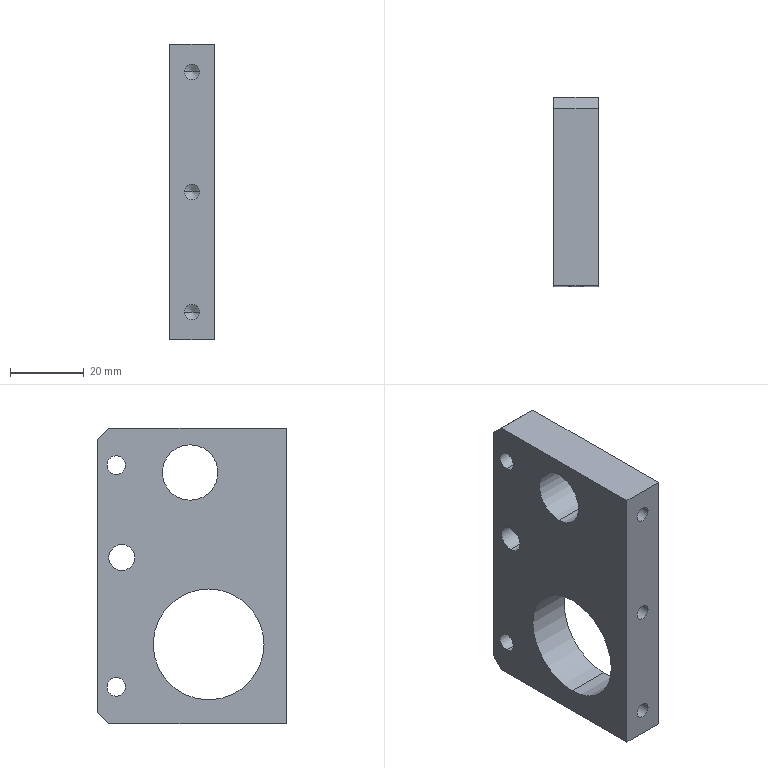Component | SolidWorks | A039-1 | 1 solid | 30 faces | box 12 x 51 x 80 mm | volume 36883 mm3 | cylinder 16 | plane 8 | cone 6 | commonest cylinder face diameters 4.2 x6 5 x4 7 x2 30 x2 15 x2
build123d program:
from build123d import *

# Parameters (mm, degrees)
SKETCH1_W             = 80
SKETCH1_H             = 51
BOSS_EXTRUDE1_DEPTH   = 12
CHAMFER1_SIZE         = 3
M5_TAPPED_HOLE1_D     = 4.2
M5_TAPPED_HOLE1_DEPTH = 10
M5_TAPPED_HOLE1_TIP   = 1.262
SKETCH6_R             = 7.5
SKETCH6_R_2           = 15
CUT_EXTRUDE1_DEPTH    = 20
M5_TAPPED_HOLE2_D     = 4.2
M5_TAPPED_HOLE2_DEPTH = 10
M5_TAPPED_HOLE2_TIP   = 1.262
M5_TAPPED_HOLE3_D     = 5
M8X1_0_TAPPED_HOLE1_D = 7


with BuildPart() as part:
    # Sketch1 → Boss-Extrude1 (new body)
    with BuildSketch(Plane.XY):
        Rectangle(SKETCH1_W, SKETCH1_H)
    extrude(amount=BOSS_EXTRUDE1_DEPTH)

    # Chamfer1
    chamfer1_edges = [part.edges().sort_by_distance(p)[0] for p in [
        (-40, 25.5, 6),
        (40, 25.5, 6),
    ]]
    chamfer(chamfer1_edges, length=CHAMFER1_SIZE)

    # M5 Tapped Hole1
    with Locations(Plane(origin=(0, -25.5, 0), x_dir=(-1, 0, 0), z_dir=(0, -1, 0))):
        with Locations((32.5, -6), (-32.5, -6)):
            Hole(M5_TAPPED_HOLE1_D / 2, depth=M5_TAPPED_HOLE1_DEPTH)
            with Locations((0, 0, -(M5_TAPPED_HOLE1_DEPTH + M5_TAPPED_HOLE1_TIP / 2))):  # 118° drill point
                Cone(0, M5_TAPPED_HOLE1_D / 2, M5_TAPPED_HOLE1_TIP, mode=Mode.SUBTRACT)

    # Sketch6 → Cut-Extrude1 (cut)
    with BuildSketch(Plane(origin=(0, 0, 0), x_dir=(-1, 0, 0), z_dir=(0, 0, -1))):
        with Locations((28, 0.5)):
            Circle(SKETCH6_R)
        with Locations((-18.5, -4.5)):
            Circle(SKETCH6_R_2)
    extrude(amount=-CUT_EXTRUDE1_DEPTH, mode=Mode.SUBTRACT)

    # M5 Tapped Hole2
    with Locations(Plane(origin=(0, -25.5, 0), x_dir=(-1, 0, 0), z_dir=(0, -1, 0))):
        with Locations((0, -6)):
            Hole(M5_TAPPED_HOLE2_D / 2, depth=M5_TAPPED_HOLE2_DEPTH)
            with Locations((0, 0, -(M5_TAPPED_HOLE2_DEPTH + M5_TAPPED_HOLE2_TIP / 2))):  # 118° drill point
                Cone(0, M5_TAPPED_HOLE2_D / 2, M5_TAPPED_HOLE2_TIP, mode=Mode.SUBTRACT)

    # M5 Tapped Hole3 (through all)
    with Locations(Plane.XY.offset(12)):
        with Locations((30, 20.5), (-30, 20.5)):
            Hole(M5_TAPPED_HOLE3_D / 2)

    # M8x1.0 Tapped Hole1 (through all)
    with Locations(Plane.XY.offset(12)):
        with Locations((-5, 19)):
            Hole(M8X1_0_TAPPED_HOLE1_D / 2)


solid = part.part

# Placed as in the assembly
solid = solid.moved(Location((321.381, 25.5, 60), (0, 90, 0)))
STEP:
#1=COLOUR_RGB('',0.7922,0.8196,0.9333);
#2=FILL_AREA_STYLE_COLOUR('',#1);
#3=FILL_AREA_STYLE('',(#2));
#4=SURFACE_STYLE_FILL_AREA(#3);
#5=SURFACE_SIDE_STYLE('',(#4));
#6=SURFACE_STYLE_USAGE(.BOTH.,#5);
#7=PRESENTATION_STYLE_ASSIGNMENT((#6));
#8=CARTESIAN_POINT('',(12.653,1.752,2.697));
#9=VERTEX_POINT('',#8);
#10=CARTESIAN_POINT('',(12.653,1.752,2.421));
#11=VERTEX_POINT('',#10);
#12=CARTESIAN_POINT('',(12.653,1.752,2.559));
#13=DIRECTION('',(1.,-0.,0.));
#14=DIRECTION('',(0.,0.,-1.));
#15=AXIS2_PLACEMENT_3D('',#12,#13,#14);
#16=CIRCLE('',#15,0.1378);
#17=EDGE_CURVE('',#9,#11,#16,.T.);
#18=ORIENTED_EDGE('',*,*,#17,.F.);
#19=CARTESIAN_POINT('',(13.125,1.752,2.697));
#20=VERTEX_POINT('',#19);
#21=CARTESIAN_POINT('',(13.125,1.752,2.697));
#22=DIRECTION('',(1.,-0.,0.));
#23=VECTOR('',#22,39.37);
#24=LINE('',#21,#23);
#25=EDGE_CURVE('',#9,#20,#24,.T.);
#26=ORIENTED_EDGE('',*,*,#25,.T.);
#27=CARTESIAN_POINT('',(13.125,1.752,2.421));
#28=VERTEX_POINT('',#27);
#29=CARTESIAN_POINT('',(13.125,1.752,2.559));
#30=DIRECTION('',(1.,-0.,0.));
#31=DIRECTION('',(0.,0.,-1.));
#32=AXIS2_PLACEMENT_3D('',#29,#30,#31);
#33=CIRCLE('',#32,0.1378);
#34=EDGE_CURVE('',#20,#28,#33,.T.);
#35=ORIENTED_EDGE('',*,*,#34,.T.);
#36=CARTESIAN_POINT('',(13.125,1.752,2.421));
#37=DIRECTION('',(1.,-0.,0.));
#38=VECTOR('',#37,39.37);
#39=LINE('',#36,#38);
#40=EDGE_CURVE('',#11,#28,#39,.T.);
#41=ORIENTED_EDGE('',*,*,#40,.F.);
#42=EDGE_LOOP('',(#18,#26,#35,#41));
#43=FACE_OUTER_BOUND('',#42,.T.);
#44=CARTESIAN_POINT('',(13.125,1.752,2.559));
#45=DIRECTION('',(1.,-0.,0.));
#46=DIRECTION('',(0.,0.,-1.));
#47=AXIS2_PLACEMENT_3D('',#44,#45,#46);
#48=CYLINDRICAL_SURFACE('',#47,0.1378);
#49=ADVANCED_FACE('',(#43),#48,.F.);
#50=CARTESIAN_POINT('',(12.653,1.811,1.28));
#51=VERTEX_POINT('',#50);
#52=CARTESIAN_POINT('',(12.653,1.811,1.083));
#53=VERTEX_POINT('',#52);
#54=CARTESIAN_POINT('',(12.653,1.811,1.181));
#55=DIRECTION('',(1.,-0.,0.));
#56=DIRECTION('',(0.,0.,-1.));
#57=AXIS2_PLACEMENT_3D('',#54,#55,#56);
#58=CIRCLE('',#57,0.09843);
#59=EDGE_CURVE('',#51,#53,#58,.T.);
#60=ORIENTED_EDGE('',*,*,#59,.F.);
#61=CARTESIAN_POINT('',(13.125,1.811,1.28));
#62=VERTEX_POINT('',#61);
#63=CARTESIAN_POINT('',(13.125,1.811,1.28));
#64=DIRECTION('',(1.,-0.,0.));
#65=VECTOR('',#64,39.37);
#66=LINE('',#63,#65);
#67=EDGE_CURVE('',#51,#62,#66,.T.);
#68=ORIENTED_EDGE('',*,*,#67,.T.);
#69=CARTESIAN_POINT('',(13.125,1.811,1.083));
#70=VERTEX_POINT('',#69);
#71=CARTESIAN_POINT('',(13.125,1.811,1.181));
#72=DIRECTION('',(1.,-0.,0.));
#73=DIRECTION('',(0.,0.,-1.));
#74=AXIS2_PLACEMENT_3D('',#71,#72,#73);
#75=CIRCLE('',#74,0.09843);
#76=EDGE_CURVE('',#62,#70,#75,.T.);
#77=ORIENTED_EDGE('',*,*,#76,.T.);
#78=CARTESIAN_POINT('',(13.125,1.811,1.083));
#79=DIRECTION('',(1.,-0.,0.));
#80=VECTOR('',#79,39.37);
#81=LINE('',#78,#80);
#82=EDGE_CURVE('',#53,#70,#81,.T.);
#83=ORIENTED_EDGE('',*,*,#82,.F.);
#84=EDGE_LOOP('',(#60,#68,#77,#83));
#85=FACE_OUTER_BOUND('',#84,.T.);
#86=CARTESIAN_POINT('',(13.125,1.811,1.181));
#87=DIRECTION('',(1.,-0.,0.));
#88=DIRECTION('',(0.,0.,-1.));
#89=AXIS2_PLACEMENT_3D('',#86,#87,#88);
#90=CYLINDRICAL_SURFACE('',#89,0.09843);
#91=ADVANCED_FACE('',(#85),#90,.F.);
#92=CARTESIAN_POINT('',(12.653,1.811,3.642));
#93=VERTEX_POINT('',#92);
#94=CARTESIAN_POINT('',(12.653,1.811,3.445));
#95=VERTEX_POINT('',#94);
#96=CARTESIAN_POINT('',(12.653,1.811,3.543));
#97=DIRECTION('',(1.,-0.,0.));
#98=DIRECTION('',(0.,0.,-1.));
#99=AXIS2_PLACEMENT_3D('',#96,#97,#98);
#100=CIRCLE('',#99,0.09843);
#101=EDGE_CURVE('',#93,#95,#100,.T.);
#102=ORIENTED_EDGE('',*,*,#101,.F.);
#103=CARTESIAN_POINT('',(13.125,1.811,3.642));
#104=VERTEX_POINT('',#103);
#105=CARTESIAN_POINT('',(13.125,1.811,3.642));
#106=DIRECTION('',(1.,-0.,0.));
#107=VECTOR('',#106,39.37);
#108=LINE('',#105,#107);
#109=EDGE_CURVE('',#93,#104,#108,.T.);
#110=ORIENTED_EDGE('',*,*,#109,.T.);
#111=CARTESIAN_POINT('',(13.125,1.811,3.445));
#112=VERTEX_POINT('',#111);
#113=CARTESIAN_POINT('',(13.125,1.811,3.543));
#114=DIRECTION('',(1.,-0.,0.));
#115=DIRECTION('',(0.,0.,-1.));
#116=AXIS2_PLACEMENT_3D('',#113,#114,#115);
#117=CIRCLE('',#116,0.09843);
#118=EDGE_CURVE('',#104,#112,#117,.T.);
#119=ORIENTED_EDGE('',*,*,#118,.T.);
#120=CARTESIAN_POINT('',(13.125,1.811,3.445));
#121=DIRECTION('',(1.,-0.,0.));
#122=VECTOR('',#121,39.37);
#123=LINE('',#120,#122);
#124=EDGE_CURVE('',#95,#112,#123,.T.);
#125=ORIENTED_EDGE('',*,*,#124,.F.);
#126=EDGE_LOOP('',(#102,#110,#119,#125));
#127=FACE_OUTER_BOUND('',#126,.T.);
#128=CARTESIAN_POINT('',(13.125,1.811,3.543));
#129=DIRECTION('',(1.,-0.,0.));
#130=DIRECTION('',(0.,0.,-1.));
#131=AXIS2_PLACEMENT_3D('',#128,#129,#130);
#132=CYLINDRICAL_SURFACE('',#131,0.09843);
#133=ADVANCED_FACE('',(#127),#132,.F.);
#134=CARTESIAN_POINT('',(12.972,0.3937,2.362));
#135=VERTEX_POINT('',#134);
#136=CARTESIAN_POINT('',(12.806,0.3937,2.362));
#137=VERTEX_POINT('',#136);
#138=CARTESIAN_POINT('',(12.889,0.3937,2.362));
#139=DIRECTION('',(-0.,-1.,-0.));
#140=DIRECTION('',(-1.,0.,0.));
#141=AXIS2_PLACEMENT_3D('',#138,#139,#140);
#142=CIRCLE('',#141,0.08268);
#143=EDGE_CURVE('',#135,#137,#142,.T.);
#144=ORIENTED_EDGE('',*,*,#143,.F.);
#145=CARTESIAN_POINT('',(12.972,-0.,2.362));
#146=VERTEX_POINT('',#145);
#147=CARTESIAN_POINT('',(12.972,-0.,2.362));
#148=DIRECTION('',(-0.,-1.,-0.));
#149=VECTOR('',#148,39.37);
#150=LINE('',#147,#149);
#151=EDGE_CURVE('',#135,#146,#150,.T.);
#152=ORIENTED_EDGE('',*,*,#151,.T.);
#153=CARTESIAN_POINT('',(12.806,-0.,2.362));
#154=VERTEX_POINT('',#153);
#155=CARTESIAN_POINT('',(12.889,-0.,2.362));
#156=DIRECTION('',(-0.,-1.,-0.));
#157=DIRECTION('',(-1.,0.,0.));
#158=AXIS2_PLACEMENT_3D('',#155,#156,#157);
#159=CIRCLE('',#158,0.08268);
#160=EDGE_CURVE('',#146,#154,#159,.T.);
#161=ORIENTED_EDGE('',*,*,#160,.T.);
#162=CARTESIAN_POINT('',(12.806,-0.,2.362));
#163=DIRECTION('',(-0.,-1.,-0.));
#164=VECTOR('',#163,39.37);
#165=LINE('',#162,#164);
#166=EDGE_CURVE('',#137,#154,#165,.T.);
#167=ORIENTED_EDGE('',*,*,#166,.F.);
#168=EDGE_LOOP('',(#144,#152,#161,#167));
#169=FACE_OUTER_BOUND('',#168,.T.);
#170=CARTESIAN_POINT('',(12.889,-0.,2.362));
#171=DIRECTION('',(-0.,-1.,-0.));
#172=DIRECTION('',(-1.,0.,0.));
#173=AXIS2_PLACEMENT_3D('',#170,#171,#172);
#174=CYLINDRICAL_SURFACE('',#173,0.08268);
#175=ADVANCED_FACE('',(#169),#174,.F.);
#176=CARTESIAN_POINT('',(12.889,0.4434,2.362));
#177=VERTEX_POINT('',#176);
#178=CARTESIAN_POINT('',(12.806,0.3937,2.362));
#179=DIRECTION('',(-0.8572,-0.515,-0.));
#180=VECTOR('',#179,39.37);
#181=LINE('',#178,#180);
#182=EDGE_CURVE('',#177,#137,#181,.T.);
#183=ORIENTED_EDGE('',*,*,#182,.F.);
#184=CARTESIAN_POINT('',(12.972,0.3937,2.362));
#185=DIRECTION('',(0.8572,-0.515,0.));
#186=VECTOR('',#185,39.37);
#187=LINE('',#184,#186);
#188=EDGE_CURVE('',#177,#135,#187,.T.);
#189=ORIENTED_EDGE('',*,*,#188,.T.);
#190=ORIENTED_EDGE('',*,*,#143,.T.);
#191=EDGE_LOOP('',(#183,#189,#190));
#192=FACE_OUTER_BOUND('',#191,.T.);
#193=CARTESIAN_POINT('',(12.889,0.3937,2.362));
#194=DIRECTION('',(-0.,-1.,-0.));
#195=DIRECTION('',(-1.,0.,0.));
#196=AXIS2_PLACEMENT_3D('',#193,#194,#195);
#197=CONICAL_SURFACE('',#196,0.08268,1.03);
#198=ADVANCED_FACE('',(#192),#197,.F.);
#199=CARTESIAN_POINT('',(13.125,0.8268,2.224));
#200=VERTEX_POINT('',#199);
#201=CARTESIAN_POINT('',(13.125,0.8268,1.043));
#202=VERTEX_POINT('',#201);
#203=CARTESIAN_POINT('',(13.125,0.8268,1.634));
#204=DIRECTION('',(1.,-0.,0.));
#205=DIRECTION('',(0.,0.,-1.));
#206=AXIS2_PLACEMENT_3D('',#203,#204,#205);
#207=CIRCLE('',#206,0.5906);
#208=EDGE_CURVE('',#200,#202,#207,.T.);
#209=ORIENTED_EDGE('',*,*,#208,.T.);
#210=CARTESIAN_POINT('',(12.653,0.8268,1.043));
#211=VERTEX_POINT('',#210);
#212=CARTESIAN_POINT('',(13.44,0.8268,1.043));
#213=DIRECTION('',(-1.,0.,-0.));
#214=VECTOR('',#213,39.37);
#215=LINE('',#212,#214);
#216=EDGE_CURVE('',#202,#211,#215,.T.);
#217=ORIENTED_EDGE('',*,*,#216,.T.);
#218=CARTESIAN_POINT('',(12.653,0.8268,2.224));
#219=VERTEX_POINT('',#218);
#220=CARTESIAN_POINT('',(12.653,0.8268,1.634));
#221=DIRECTION('',(-1.,0.,-0.));
#222=DIRECTION('',(0.,-0.,1.));
#223=AXIS2_PLACEMENT_3D('',#220,#221,#222);
#224=CIRCLE('',#223,0.5906);
#225=EDGE_CURVE('',#211,#219,#224,.T.);
#226=ORIENTED_EDGE('',*,*,#225,.T.);
#227=CARTESIAN_POINT('',(13.44,0.8268,2.224));
#228=DIRECTION('',(-1.,0.,-0.));
#229=VECTOR('',#228,39.37);
#230=LINE('',#227,#229);
#231=EDGE_CURVE('',#200,#219,#230,.T.);
#232=ORIENTED_EDGE('',*,*,#231,.F.);
#233=EDGE_LOOP('',(#209,#217,#226,#232));
#234=FACE_OUTER_BOUND('',#233,.T.);
#235=CARTESIAN_POINT('',(13.44,0.8268,1.634));
#236=DIRECTION('',(-1.,0.,-0.));
#237=DIRECTION('',(0.,-0.,1.));
#238=AXIS2_PLACEMENT_3D('',#235,#236,#237);
#239=CYLINDRICAL_SURFACE('',#238,0.5906);
#240=ADVANCED_FACE('',(#234),#239,.F.);
#241=CARTESIAN_POINT('',(13.125,1.024,3.76));
#242=VERTEX_POINT('',#241);
#243=CARTESIAN_POINT('',(13.125,1.024,3.169));
#244=VERTEX_POINT('',#243);
#245=CARTESIAN_POINT('',(13.125,1.024,3.465));
#246=DIRECTION('',(1.,-0.,0.));
#247=DIRECTION('',(0.,0.,-1.));
#248=AXIS2_PLACEMENT_3D('',#245,#246,#247);
#249=CIRCLE('',#248,0.2953);
#250=EDGE_CURVE('',#242,#244,#249,.T.);
#251=ORIENTED_EDGE('',*,*,#250,.T.);
#252=CARTESIAN_POINT('',(12.653,1.024,3.169));
#253=VERTEX_POINT('',#252);
#254=CARTESIAN_POINT('',(13.44,1.024,3.169));
#255=DIRECTION('',(-1.,0.,-0.));
#256=VECTOR('',#255,39.37);
#257=LINE('',#254,#256);
#258=EDGE_CURVE('',#244,#253,#257,.T.);
#259=ORIENTED_EDGE('',*,*,#258,.T.);
#260=CARTESIAN_POINT('',(12.653,1.024,3.76));
#261=VERTEX_POINT('',#260);
#262=CARTESIAN_POINT('',(12.653,1.024,3.465));
#263=DIRECTION('',(-1.,0.,-0.));
#264=DIRECTION('',(0.,0.,1.));
#265=AXIS2_PLACEMENT_3D('',#262,#263,#264);
#266=CIRCLE('',#265,0.2953);
#267=EDGE_CURVE('',#253,#261,#266,.T.);
#268=ORIENTED_EDGE('',*,*,#267,.T.);
#269=CARTESIAN_POINT('',(13.44,1.024,3.76));
#270=DIRECTION('',(-1.,0.,-0.));
#271=VECTOR('',#270,39.37);
#272=LINE('',#269,#271);
#273=EDGE_CURVE('',#242,#261,#272,.T.);
#274=ORIENTED_EDGE('',*,*,#273,.F.);
#275=EDGE_LOOP('',(#251,#259,#268,#274));
#276=FACE_OUTER_BOUND('',#275,.T.);
#277=CARTESIAN_POINT('',(13.44,1.024,3.465));
#278=DIRECTION('',(-1.,0.,-0.));
#279=DIRECTION('',(0.,0.,1.));
#280=AXIS2_PLACEMENT_3D('',#277,#278,#279);
#281=CYLINDRICAL_SURFACE('',#280,0.2953);
#282=ADVANCED_FACE('',(#276),#281,.F.);
#283=CARTESIAN_POINT('',(12.972,0.3937,3.642));
#284=VERTEX_POINT('',#283);
#285=CARTESIAN_POINT('',(12.806,0.3937,3.642));
#286=VERTEX_POINT('',#285);
#287=CARTESIAN_POINT('',(12.889,0.3937,3.642));
#288=DIRECTION('',(-0.,-1.,-0.));
#289=DIRECTION('',(-1.,0.,0.));
#290=AXIS2_PLACEMENT_3D('',#287,#288,#289);
#291=CIRCLE('',#290,0.08268);
#292=EDGE_CURVE('',#284,#286,#291,.T.);
#293=ORIENTED_EDGE('',*,*,#292,.F.);
#294=CARTESIAN_POINT('',(12.972,-0.,3.642));
#295=VERTEX_POINT('',#294);
#296=CARTESIAN_POINT('',(12.972,-0.,3.642));
#297=DIRECTION('',(-0.,-1.,-0.));
#298=VECTOR('',#297,39.37);
#299=LINE('',#296,#298);
#300=EDGE_CURVE('',#284,#295,#299,.T.);
#301=ORIENTED_EDGE('',*,*,#300,.T.);
#302=CARTESIAN_POINT('',(12.806,-0.,3.642));
#303=VERTEX_POINT('',#302);
#304=CARTESIAN_POINT('',(12.889,-0.,3.642));
#305=DIRECTION('',(-0.,-1.,-0.));
#306=DIRECTION('',(-1.,0.,0.));
#307=AXIS2_PLACEMENT_3D('',#304,#305,#306);
#308=CIRCLE('',#307,0.08268);
#309=EDGE_CURVE('',#295,#303,#308,.T.);
#310=ORIENTED_EDGE('',*,*,#309,.T.);
#311=CARTESIAN_POINT('',(12.806,-0.,3.642));
#312=DIRECTION('',(-0.,-1.,-0.));
#313=VECTOR('',#312,39.37);
#314=LINE('',#311,#313);
#315=EDGE_CURVE('',#286,#303,#314,.T.);
#316=ORIENTED_EDGE('',*,*,#315,.F.);
#317=EDGE_LOOP('',(#293,#301,#310,#316));
#318=FACE_OUTER_BOUND('',#317,.T.);
#319=CARTESIAN_POINT('',(12.889,-0.,3.642));
#320=DIRECTION('',(-0.,-1.,-0.));
#321=DIRECTION('',(-1.,0.,0.));
#322=AXIS2_PLACEMENT_3D('',#319,#320,#321);
#323=CYLINDRICAL_SURFACE('',#322,0.08268);
#324=ADVANCED_FACE('',(#318),#323,.F.);
#325=CARTESIAN_POINT('',(12.889,0.4434,3.642));
#326=VERTEX_POINT('',#325);
#327=CARTESIAN_POINT('',(12.806,0.3937,3.642));
#328=DIRECTION('',(-0.8572,-0.515,-0.));
#329=VECTOR('',#328,39.37);
#330=LINE('',#327,#329);
#331=EDGE_CURVE('',#326,#286,#330,.T.);
#332=ORIENTED_EDGE('',*,*,#331,.F.);
#333=CARTESIAN_POINT('',(12.972,0.3937,3.642));
#334=DIRECTION('',(0.8572,-0.515,0.));
#335=VECTOR('',#334,39.37);
#336=LINE('',#333,#335);
#337=EDGE_CURVE('',#326,#284,#336,.T.);
#338=ORIENTED_EDGE('',*,*,#337,.T.);
#339=ORIENTED_EDGE('',*,*,#292,.T.);
#340=EDGE_LOOP('',(#332,#338,#339));
#341=FACE_OUTER_BOUND('',#340,.T.);
#342=CARTESIAN_POINT('',(12.889,0.3937,3.642));
#343=DIRECTION('',(-0.,-1.,-0.));
#344=DIRECTION('',(-1.,0.,0.));
#345=AXIS2_PLACEMENT_3D('',#342,#343,#344);
#346=CONICAL_SURFACE('',#345,0.08268,1.03);
#347=ADVANCED_FACE('',(#341),#346,.F.);
#348=CARTESIAN_POINT('',(12.972,0.3937,1.083));
#349=VERTEX_POINT('',#348);
#350=CARTESIAN_POINT('',(12.806,0.3937,1.083));
#351=VERTEX_POINT('',#350);
#352=CARTESIAN_POINT('',(12.889,0.3937,1.083));
#353=DIRECTION('',(-0.,-1.,-0.));
#354=DIRECTION('',(-1.,0.,0.));
#355=AXIS2_PLACEMENT_3D('',#352,#353,#354);
#356=CIRCLE('',#355,0.08268);
#357=EDGE_CURVE('',#349,#351,#356,.T.);
#358=ORIENTED_EDGE('',*,*,#357,.F.);
#359=CARTESIAN_POINT('',(12.972,-0.,1.083));
#360=VERTEX_POINT('',#359);
#361=CARTESIAN_POINT('',(12.972,-0.,1.083));
#362=DIRECTION('',(-0.,-1.,-0.));
#363=VECTOR('',#362,39.37);
#364=LINE('',#361,#363);
#365=EDGE_CURVE('',#349,#360,#364,.T.);
#366=ORIENTED_EDGE('',*,*,#365,.T.);
#367=CARTESIAN_POINT('',(12.806,-0.,1.083));
#368=VERTEX_POINT('',#367);
#369=CARTESIAN_POINT('',(12.889,-0.,1.083));
#370=DIRECTION('',(-0.,-1.,-0.));
#371=DIRECTION('',(-1.,0.,0.));
#372=AXIS2_PLACEMENT_3D('',#369,#370,#371);
#373=CIRCLE('',#372,0.08268);
#374=EDGE_CURVE('',#360,#368,#373,.T.);
#375=ORIENTED_EDGE('',*,*,#374,.T.);
#376=CARTESIAN_POINT('',(12.806,-0.,1.083));
#377=DIRECTION('',(-0.,-1.,-0.));
#378=VECTOR('',#377,39.37);
#379=LINE('',#376,#378);
#380=EDGE_CURVE('',#351,#368,#379,.T.);
#381=ORIENTED_EDGE('',*,*,#380,.F.);
#382=EDGE_LOOP('',(#358,#366,#375,#381));
#383=FACE_OUTER_BOUND('',#382,.T.);
#384=CARTESIAN_POINT('',(12.889,-0.,1.083));
#385=DIRECTION('',(-0.,-1.,-0.));
#386=DIRECTION('',(-1.,0.,0.));
#387=AXIS2_PLACEMENT_3D('',#384,#385,#386);
#388=CYLINDRICAL_SURFACE('',#387,0.08268);
#389=ADVANCED_FACE('',(#383),#388,.F.);
#390=CARTESIAN_POINT('',(12.889,0.4434,1.083));
#391=VERTEX_POINT('',#390);
#392=CARTESIAN_POINT('',(12.806,0.3937,1.083));
#393=DIRECTION('',(-0.8572,-0.515,-0.));
#394=VECTOR('',#393,39.37);
#395=LINE('',#392,#394);
#396=EDGE_CURVE('',#391,#351,#395,.T.);
#397=ORIENTED_EDGE('',*,*,#396,.F.);
#398=CARTESIAN_POINT('',(12.972,0.3937,1.083));
#399=DIRECTION('',(0.8572,-0.515,0.));
#400=VECTOR('',#399,39.37);
#401=LINE('',#398,#400);
#402=EDGE_CURVE('',#391,#349,#401,.T.);
#403=ORIENTED_EDGE('',*,*,#402,.T.);
#404=ORIENTED_EDGE('',*,*,#357,.T.);
#405=EDGE_LOOP('',(#397,#403,#404));
#406=FACE_OUTER_BOUND('',#405,.T.);
#407=CARTESIAN_POINT('',(12.889,0.3937,1.083));
#408=DIRECTION('',(-0.,-1.,-0.));
#409=DIRECTION('',(-1.,0.,0.));
#410=AXIS2_PLACEMENT_3D('',#407,#408,#409);
#411=CONICAL_SURFACE('',#410,0.08268,1.03);
#412=ADVANCED_FACE('',(#406),#411,.F.);
#413=CARTESIAN_POINT('',(12.653,-0.,0.7874));
#414=VERTEX_POINT('',#413);
#415=CARTESIAN_POINT('',(12.653,1.89,0.7874));
#416=VERTEX_POINT('',#415);
#417=CARTESIAN_POINT('',(12.653,2.008,0.7874));
#418=DIRECTION('',(0.,1.,0.));
#419=VECTOR('',#418,39.37);
#420=LINE('',#417,#419);
#421=EDGE_CURVE('',#414,#416,#420,.T.);
#422=ORIENTED_EDGE('',*,*,#421,.T.);
#423=CARTESIAN_POINT('',(13.125,1.89,0.7874));
#424=VERTEX_POINT('',#423);
#425=CARTESIAN_POINT('',(13.125,1.89,0.7874));
#426=DIRECTION('',(1.,-0.,0.));
#427=VECTOR('',#426,39.37);
#428=LINE('',#425,#427);
#429=EDGE_CURVE('',#416,#424,#428,.T.);
#430=ORIENTED_EDGE('',*,*,#429,.T.);
#431=CARTESIAN_POINT('',(13.125,-0.,0.7874));
#432=VERTEX_POINT('',#431);
#433=CARTESIAN_POINT('',(13.125,2.008,0.7874));
#434=DIRECTION('',(0.,1.,0.));
#435=VECTOR('',#434,39.37);
#436=LINE('',#433,#435);
#437=EDGE_CURVE('',#432,#424,#436,.T.);
#438=ORIENTED_EDGE('',*,*,#437,.F.);
#439=CARTESIAN_POINT('',(13.125,-0.,0.7874));
#440=DIRECTION('',(-1.,0.,-0.));
#441=VECTOR('',#440,39.37);
#442=LINE('',#439,#441);
#443=EDGE_CURVE('',#432,#414,#442,.T.);
#444=ORIENTED_EDGE('',*,*,#443,.T.);
#445=EDGE_LOOP('',(#422,#430,#438,#444));
#446=FACE_OUTER_BOUND('',#445,.T.);
#447=CARTESIAN_POINT('',(13.125,2.008,0.7874));
#448=DIRECTION('',(-0.,-0.,1.));
#449=DIRECTION('',(1.,-0.,0.));
#450=AXIS2_PLACEMENT_3D('',#447,#448,#449);
#451=PLANE('',#450);
#452=ADVANCED_FACE('',(#446),#451,.F.);
#453=CARTESIAN_POINT('',(13.125,2.008,0.9055));
#454=VERTEX_POINT('',#453);
#455=CARTESIAN_POINT('',(13.125,2.008,3.819));
#456=VERTEX_POINT('',#455);
#457=CARTESIAN_POINT('',(13.125,2.008,3.937));
#458=DIRECTION('',(-0.,-0.,1.));
#459=VECTOR('',#458,39.37);
#460=LINE('',#457,#459);
#461=EDGE_CURVE('',#454,#456,#460,.T.);
#462=ORIENTED_EDGE('',*,*,#461,.F.);
#463=CARTESIAN_POINT('',(12.653,2.008,0.9055));
#464=VERTEX_POINT('',#463);
#465=CARTESIAN_POINT('',(13.125,2.008,0.9055));
#466=DIRECTION('',(-1.,0.,-0.));
#467=VECTOR('',#466,39.37);
#468=LINE('',#465,#467);
#469=EDGE_CURVE('',#454,#464,#468,.T.);
#470=ORIENTED_EDGE('',*,*,#469,.T.);
#471=CARTESIAN_POINT('',(12.653,2.008,3.819));
#472=VERTEX_POINT('',#471);
#473=CARTESIAN_POINT('',(12.653,2.008,3.937));
#474=DIRECTION('',(-0.,-0.,1.));
#475=VECTOR('',#474,39.37);
#476=LINE('',#473,#475);
#477=EDGE_CURVE('',#464,#472,#476,.T.);
#478=ORIENTED_EDGE('',*,*,#477,.T.);
#479=CARTESIAN_POINT('',(13.125,2.008,3.819));
#480=DIRECTION('',(1.,-0.,0.));
#481=VECTOR('',#480,39.37);
#482=LINE('',#479,#481);
#483=EDGE_CURVE('',#472,#456,#482,.T.);
#484=ORIENTED_EDGE('',*,*,#483,.T.);
#485=EDGE_LOOP('',(#462,#470,#478,#484));
#486=FACE_OUTER_BOUND('',#485,.T.);
#487=CARTESIAN_POINT('',(13.125,2.008,3.937));
#488=DIRECTION('',(-0.,-1.,-0.));
#489=DIRECTION('',(-1.,0.,-0.));
#490=AXIS2_PLACEMENT_3D('',#487,#488,#489);
#491=PLANE('',#490);
#492=ADVANCED_FACE('',(#486),#491,.F.);
#493=CARTESIAN_POINT('',(13.125,1.89,3.937));
#494=VERTEX_POINT('',#493);
#495=CARTESIAN_POINT('',(13.125,-0.,3.937));
#496=VERTEX_POINT('',#495);
#497=CARTESIAN_POINT('',(13.125,2.008,3.937));
#498=DIRECTION('',(-0.,-1.,-0.));
#499=VECTOR('',#498,39.37);
#500=LINE('',#497,#499);
#501=EDGE_CURVE('',#494,#496,#500,.T.);
#502=ORIENTED_EDGE('',*,*,#501,.F.);
#503=CARTESIAN_POINT('',(12.653,1.89,3.937));
#504=VERTEX_POINT('',#503);
#505=CARTESIAN_POINT('',(13.125,1.89,3.937));
#506=DIRECTION('',(-1.,0.,-0.));
#507=VECTOR('',#506,39.37);
#508=LINE('',#505,#507);
#509=EDGE_CURVE('',#494,#504,#508,.T.);
#510=ORIENTED_EDGE('',*,*,#509,.T.);
#511=CARTESIAN_POINT('',(12.653,-0.,3.937));
#512=VERTEX_POINT('',#511);
#513=CARTESIAN_POINT('',(12.653,2.008,3.937));
#514=DIRECTION('',(-0.,-1.,-0.));
#515=VECTOR('',#514,39.37);
#516=LINE('',#513,#515);
#517=EDGE_CURVE('',#504,#512,#516,.T.);
#518=ORIENTED_EDGE('',*,*,#517,.T.);
#519=CARTESIAN_POINT('',(13.125,-0.,3.937));
#520=DIRECTION('',(-1.,0.,-0.));
#521=VECTOR('',#520,39.37);
#522=LINE('',#519,#521);
#523=EDGE_CURVE('',#496,#512,#522,.T.);
#524=ORIENTED_EDGE('',*,*,#523,.F.);
#525=EDGE_LOOP('',(#502,#510,#518,#524));
#526=FACE_OUTER_BOUND('',#525,.T.);
#527=CARTESIAN_POINT('',(13.125,2.008,3.937));
#528=DIRECTION('',(0.,0.,-1.));
#529=DIRECTION('',(0.,1.,0.));
#530=AXIS2_PLACEMENT_3D('',#527,#528,#529);
#531=PLANE('',#530);
#532=ADVANCED_FACE('',(#526),#531,.F.);
#533=CARTESIAN_POINT('',(12.889,-0.,2.362));
#534=DIRECTION('',(-0.,-1.,-0.));
#535=DIRECTION('',(-1.,0.,0.));
#536=AXIS2_PLACEMENT_3D('',#533,#534,#535);
#537=CIRCLE('',#536,0.08268);
#538=EDGE_CURVE('',#154,#146,#537,.T.);
#539=ORIENTED_EDGE('',*,*,#538,.F.);
#540=ORIENTED_EDGE('',*,*,#160,.F.);
#541=EDGE_LOOP('',(#539,#540));
#542=FACE_BOUND('',#541,.T.);
#543=CARTESIAN_POINT('',(12.889,-0.,3.642));
#544=DIRECTION('',(-0.,-1.,-0.));
#545=DIRECTION('',(-1.,0.,0.));
#546=AXIS2_PLACEMENT_3D('',#543,#544,#545);
#547=CIRCLE('',#546,0.08268);
#548=EDGE_CURVE('',#303,#295,#547,.T.);
#549=ORIENTED_EDGE('',*,*,#548,.F.);
#550=ORIENTED_EDGE('',*,*,#309,.F.);
#551=EDGE_LOOP('',(#549,#550));
#552=FACE_BOUND('',#551,.T.);
#553=CARTESIAN_POINT('',(12.889,-0.,1.083));
#554=DIRECTION('',(-0.,-1.,-0.));
#555=DIRECTION('',(-1.,0.,0.));
#556=AXIS2_PLACEMENT_3D('',#553,#554,#555);
#557=CIRCLE('',#556,0.08268);
#558=EDGE_CURVE('',#368,#360,#557,.T.);
#559=ORIENTED_EDGE('',*,*,#558,.F.);
#560=ORIENTED_EDGE('',*,*,#374,.F.);
#561=EDGE_LOOP('',(#559,#560));
#562=FACE_BOUND('',#561,.T.);
#563=CARTESIAN_POINT('',(12.653,-0.,3.937));
#564=DIRECTION('',(0.,0.,-1.));
#565=VECTOR('',#564,39.37);
#566=LINE('',#563,#565);
#567=EDGE_CURVE('',#512,#414,#566,.T.);
#568=ORIENTED_EDGE('',*,*,#567,.T.);
#569=ORIENTED_EDGE('',*,*,#443,.F.);
#570=CARTESIAN_POINT('',(13.125,-0.,3.937));
#571=DIRECTION('',(0.,0.,-1.));
#572=VECTOR('',#571,39.37);
#573=LINE('',#570,#572);
#574=EDGE_CURVE('',#496,#432,#573,.T.);
#575=ORIENTED_EDGE('',*,*,#574,.F.);
#576=ORIENTED_EDGE('',*,*,#523,.T.);
#577=EDGE_LOOP('',(#568,#569,#575,#576));
#578=FACE_OUTER_BOUND('',#577,.T.);
#579=CARTESIAN_POINT('',(13.125,-0.,3.937));
#580=DIRECTION('',(0.,1.,0.));
#581=DIRECTION('',(1.,-0.,0.));
#582=AXIS2_PLACEMENT_3D('',#579,#580,#581);
#583=PLANE('',#582);
#584=ADVANCED_FACE('',(#542,#552,#562,#578),#583,.F.);
#585=CARTESIAN_POINT('',(13.125,1.752,2.559));
#586=DIRECTION('',(1.,-0.,0.));
#587=DIRECTION('',(0.,0.,-1.));
#588=AXIS2_PLACEMENT_3D('',#585,#586,#587);
#589=CIRCLE('',#588,0.1378);
#590=EDGE_CURVE('',#28,#20,#589,.T.);
#591=ORIENTED_EDGE('',*,*,#590,.F.);
#592=ORIENTED_EDGE('',*,*,#34,.F.);
#593=EDGE_LOOP('',(#591,#592));
#594=FACE_BOUND('',#593,.T.);
#595=CARTESIAN_POINT('',(13.125,1.811,1.181));
#596=DIRECTION('',(1.,-0.,0.));
#597=DIRECTION('',(0.,0.,-1.));
#598=AXIS2_PLACEMENT_3D('',#595,#596,#597);
#599=CIRCLE('',#598,0.09843);
#600=EDGE_CURVE('',#70,#62,#599,.T.);
#601=ORIENTED_EDGE('',*,*,#600,.F.);
#602=ORIENTED_EDGE('',*,*,#76,.F.);
#603=EDGE_LOOP('',(#601,#602));
#604=FACE_BOUND('',#603,.T.);
#605=CARTESIAN_POINT('',(13.125,1.811,3.543));
#606=DIRECTION('',(1.,-0.,0.));
#607=DIRECTION('',(0.,0.,-1.));
#608=AXIS2_PLACEMENT_3D('',#605,#606,#607);
#609=CIRCLE('',#608,0.09843);
#610=EDGE_CURVE('',#112,#104,#609,.T.);
#611=ORIENTED_EDGE('',*,*,#610,.F.);
#612=ORIENTED_EDGE('',*,*,#118,.F.);
#613=EDGE_LOOP('',(#611,#612));
#614=FACE_BOUND('',#613,.T.);
#615=ORIENTED_EDGE('',*,*,#208,.F.);
#616=CARTESIAN_POINT('',(13.125,0.8268,1.634));
#617=DIRECTION('',(1.,-0.,0.));
#618=DIRECTION('',(0.,0.,-1.));
#619=AXIS2_PLACEMENT_3D('',#616,#617,#618);
#620=CIRCLE('',#619,0.5906);
#621=EDGE_CURVE('',#202,#200,#620,.T.);
#622=ORIENTED_EDGE('',*,*,#621,.F.);
#623=EDGE_LOOP('',(#615,#622));
#624=FACE_BOUND('',#623,.T.);
#625=ORIENTED_EDGE('',*,*,#250,.F.);
#626=CARTESIAN_POINT('',(13.125,1.024,3.465));
#627=DIRECTION('',(1.,-0.,0.));
#628=DIRECTION('',(0.,0.,-1.));
#629=AXIS2_PLACEMENT_3D('',#626,#627,#628);
#630=CIRCLE('',#629,0.2953);
#631=EDGE_CURVE('',#244,#242,#630,.T.);
#632=ORIENTED_EDGE('',*,*,#631,.F.);
#633=EDGE_LOOP('',(#625,#632));
#634=FACE_BOUND('',#633,.T.);
#635=ORIENTED_EDGE('',*,*,#437,.T.);
#636=CARTESIAN_POINT('',(13.125,2.234,1.132));
#637=DIRECTION('',(-0.,0.7071,0.7071));
#638=VECTOR('',#637,39.37);
#639=LINE('',#636,#638);
#640=EDGE_CURVE('',#424,#454,#639,.T.);
#641=ORIENTED_EDGE('',*,*,#640,.T.);
#642=ORIENTED_EDGE('',*,*,#461,.T.);
#643=CARTESIAN_POINT('',(13.125,2.234,3.593));
#644=DIRECTION('',(-0.,-0.7071,0.7071));
#645=VECTOR('',#644,39.37);
#646=LINE('',#643,#645);
#647=EDGE_CURVE('',#456,#494,#646,.T.);
#648=ORIENTED_EDGE('',*,*,#647,.T.);
#649=ORIENTED_EDGE('',*,*,#501,.T.);
#650=ORIENTED_EDGE('',*,*,#574,.T.);
#651=EDGE_LOOP('',(#635,#641,#642,#648,#649,#650));
#652=FACE_OUTER_BOUND('',#651,.T.);
#653=CARTESIAN_POINT('',(13.125,1.004,2.362));
#654=DIRECTION('',(1.,-0.,0.));
#655=DIRECTION('',(0.,0.,-1.));
#656=AXIS2_PLACEMENT_3D('',#653,#654,#655);
#657=PLANE('',#656);
#658=ADVANCED_FACE('',(#594,#604,#614,#624,#634,#652),#657,.T.);
#659=CARTESIAN_POINT('',(12.653,1.752,2.559));
#660=DIRECTION('',(1.,-0.,0.));
#661=DIRECTION('',(0.,0.,-1.));
#662=AXIS2_PLACEMENT_3D('',#659,#660,#661);
#663=CIRCLE('',#662,0.1378);
#664=EDGE_CURVE('',#11,#9,#663,.T.);
#665=ORIENTED_EDGE('',*,*,#664,.T.);
#666=ORIENTED_EDGE('',*,*,#17,.T.);
#667=EDGE_LOOP('',(#665,#666));
#668=FACE_BOUND('',#667,.T.);
#669=CARTESIAN_POINT('',(12.653,1.811,1.181));
#670=DIRECTION('',(1.,-0.,0.));
#671=DIRECTION('',(0.,0.,-1.));
#672=AXIS2_PLACEMENT_3D('',#669,#670,#671);
#673=CIRCLE('',#672,0.09843);
#674=EDGE_CURVE('',#53,#51,#673,.T.);
#675=ORIENTED_EDGE('',*,*,#674,.T.);
#676=ORIENTED_EDGE('',*,*,#59,.T.);
#677=EDGE_LOOP('',(#675,#676));
#678=FACE_BOUND('',#677,.T.);
#679=CARTESIAN_POINT('',(12.653,1.811,3.543));
#680=DIRECTION('',(1.,-0.,0.));
#681=DIRECTION('',(0.,0.,-1.));
#682=AXIS2_PLACEMENT_3D('',#679,#680,#681);
#683=CIRCLE('',#682,0.09843);
#684=EDGE_CURVE('',#95,#93,#683,.T.);
#685=ORIENTED_EDGE('',*,*,#684,.T.);
#686=ORIENTED_EDGE('',*,*,#101,.T.);
#687=EDGE_LOOP('',(#685,#686));
#688=FACE_BOUND('',#687,.T.);
#689=CARTESIAN_POINT('',(12.653,0.8268,1.634));
#690=DIRECTION('',(-1.,0.,-0.));
#691=DIRECTION('',(0.,-0.,1.));
#692=AXIS2_PLACEMENT_3D('',#689,#690,#691);
#693=CIRCLE('',#692,0.5906);
#694=EDGE_CURVE('',#219,#211,#693,.T.);
#695=ORIENTED_EDGE('',*,*,#694,.F.);
#696=ORIENTED_EDGE('',*,*,#225,.F.);
#697=EDGE_LOOP('',(#695,#696));
#698=FACE_BOUND('',#697,.T.);
#699=CARTESIAN_POINT('',(12.653,1.024,3.465));
#700=DIRECTION('',(-1.,0.,-0.));
#701=DIRECTION('',(0.,0.,1.));
#702=AXIS2_PLACEMENT_3D('',#699,#700,#701);
#703=CIRCLE('',#702,0.2953);
#704=EDGE_CURVE('',#261,#253,#703,.T.);
#705=ORIENTED_EDGE('',*,*,#704,.F.);
#706=ORIENTED_EDGE('',*,*,#267,.F.);
#707=EDGE_LOOP('',(#705,#706));
#708=FACE_BOUND('',#707,.T.);
#709=ORIENTED_EDGE('',*,*,#477,.F.);
#710=CARTESIAN_POINT('',(12.653,2.008,0.9055));
#711=DIRECTION('',(0.,-0.7071,-0.7071));
#712=VECTOR('',#711,39.37);
#713=LINE('',#710,#712);
#714=EDGE_CURVE('',#464,#416,#713,.T.);
#715=ORIENTED_EDGE('',*,*,#714,.T.);
#716=ORIENTED_EDGE('',*,*,#421,.F.);
#717=ORIENTED_EDGE('',*,*,#567,.F.);
#718=ORIENTED_EDGE('',*,*,#517,.F.);
#719=CARTESIAN_POINT('',(12.653,1.89,3.937));
#720=DIRECTION('',(0.,0.7071,-0.7071));
#721=VECTOR('',#720,39.37);
#722=LINE('',#719,#721);
#723=EDGE_CURVE('',#504,#472,#722,.T.);
#724=ORIENTED_EDGE('',*,*,#723,.T.);
#725=EDGE_LOOP('',(#709,#715,#716,#717,#718,#724));
#726=FACE_OUTER_BOUND('',#725,.T.);
#727=CARTESIAN_POINT('',(12.653,1.004,2.362));
#728=DIRECTION('',(1.,-0.,0.));
#729=DIRECTION('',(0.,0.,-1.));
#730=AXIS2_PLACEMENT_3D('',#727,#728,#729);
#731=PLANE('',#730);
#732=ADVANCED_FACE('',(#668,#678,#688,#698,#708,#726),#731,.F.);
#733=ORIENTED_EDGE('',*,*,#640,.F.);
#734=ORIENTED_EDGE('',*,*,#429,.F.);
#735=ORIENTED_EDGE('',*,*,#714,.F.);
#736=ORIENTED_EDGE('',*,*,#469,.F.);
#737=EDGE_LOOP('',(#733,#734,#735,#736));
#738=FACE_OUTER_BOUND('',#737,.T.);
#739=CARTESIAN_POINT('',(13.125,2.008,0.9055));
#740=DIRECTION('',(-0.,-0.7071,0.7071));
#741=DIRECTION('',(-1.,0.,-0.));
#742=AXIS2_PLACEMENT_3D('',#739,#740,#741);
#743=PLANE('',#742);
#744=ADVANCED_FACE('',(#738),#743,.F.);
#745=ORIENTED_EDGE('',*,*,#647,.F.);
#746=ORIENTED_EDGE('',*,*,#483,.F.);
#747=ORIENTED_EDGE('',*,*,#723,.F.);
#748=ORIENTED_EDGE('',*,*,#509,.F.);
#749=EDGE_LOOP('',(#745,#746,#747,#748));
#750=FACE_OUTER_BOUND('',#749,.T.);
#751=CARTESIAN_POINT('',(13.125,1.89,3.937));
#752=DIRECTION('',(0.,-0.7071,-0.7071));
#753=DIRECTION('',(-1.,0.,-0.));
#754=AXIS2_PLACEMENT_3D('',#751,#752,#753);
#755=PLANE('',#754);
#756=ADVANCED_FACE('',(#750),#755,.F.);
#757=ORIENTED_EDGE('',*,*,#402,.F.);
#758=ORIENTED_EDGE('',*,*,#396,.T.);
#759=CARTESIAN_POINT('',(12.889,0.3937,1.083));
#760=DIRECTION('',(-0.,-1.,-0.));
#761=DIRECTION('',(-1.,0.,0.));
#762=AXIS2_PLACEMENT_3D('',#759,#760,#761);
#763=CIRCLE('',#762,0.08268);
#764=EDGE_CURVE('',#351,#349,#763,.T.);
#765=ORIENTED_EDGE('',*,*,#764,.T.);
#766=EDGE_LOOP('',(#757,#758,#765));
#767=FACE_OUTER_BOUND('',#766,.T.);
#768=CARTESIAN_POINT('',(12.889,0.3937,1.083));
#769=DIRECTION('',(-0.,-1.,-0.));
#770=DIRECTION('',(-1.,0.,0.));
#771=AXIS2_PLACEMENT_3D('',#768,#769,#770);
#772=CONICAL_SURFACE('',#771,0.08268,1.03);
#773=ADVANCED_FACE('',(#767),#772,.F.);
#774=ORIENTED_EDGE('',*,*,#365,.F.);
#775=ORIENTED_EDGE('',*,*,#764,.F.);
#776=ORIENTED_EDGE('',*,*,#380,.T.);
#777=ORIENTED_EDGE('',*,*,#558,.T.);
#778=EDGE_LOOP('',(#774,#775,#776,#777));
#779=FACE_OUTER_BOUND('',#778,.T.);
#780=CARTESIAN_POINT('',(12.889,-0.,1.083));
#781=DIRECTION('',(-0.,-1.,-0.));
#782=DIRECTION('',(-1.,0.,0.));
#783=AXIS2_PLACEMENT_3D('',#780,#781,#782);
#784=CYLINDRICAL_SURFACE('',#783,0.08268);
#785=ADVANCED_FACE('',(#779),#784,.F.);
#786=ORIENTED_EDGE('',*,*,#337,.F.);
#787=ORIENTED_EDGE('',*,*,#331,.T.);
#788=CARTESIAN_POINT('',(12.889,0.3937,3.642));
#789=DIRECTION('',(-0.,-1.,-0.));
#790=DIRECTION('',(-1.,0.,0.));
#791=AXIS2_PLACEMENT_3D('',#788,#789,#790);
#792=CIRCLE('',#791,0.08268);
#793=EDGE_CURVE('',#286,#284,#792,.T.);
#794=ORIENTED_EDGE('',*,*,#793,.T.);
#795=EDGE_LOOP('',(#786,#787,#794));
#796=FACE_OUTER_BOUND('',#795,.T.);
#797=CARTESIAN_POINT('',(12.889,0.3937,3.642));
#798=DIRECTION('',(-0.,-1.,-0.));
#799=DIRECTION('',(-1.,0.,0.));
#800=AXIS2_PLACEMENT_3D('',#797,#798,#799);
#801=CONICAL_SURFACE('',#800,0.08268,1.03);
#802=ADVANCED_FACE('',(#796),#801,.F.);
#803=ORIENTED_EDGE('',*,*,#300,.F.);
#804=ORIENTED_EDGE('',*,*,#793,.F.);
#805=ORIENTED_EDGE('',*,*,#315,.T.);
#806=ORIENTED_EDGE('',*,*,#548,.T.);
#807=EDGE_LOOP('',(#803,#804,#805,#806));
#808=FACE_OUTER_BOUND('',#807,.T.);
#809=CARTESIAN_POINT('',(12.889,-0.,3.642));
#810=DIRECTION('',(-0.,-1.,-0.));
#811=DIRECTION('',(-1.,0.,0.));
#812=AXIS2_PLACEMENT_3D('',#809,#810,#811);
#813=CYLINDRICAL_SURFACE('',#812,0.08268);
#814=ADVANCED_FACE('',(#808),#813,.F.);
#815=ORIENTED_EDGE('',*,*,#258,.F.);
#816=ORIENTED_EDGE('',*,*,#631,.T.);
#817=ORIENTED_EDGE('',*,*,#273,.T.);
#818=ORIENTED_EDGE('',*,*,#704,.T.);
#819=EDGE_LOOP('',(#815,#816,#817,#818));
#820=FACE_OUTER_BOUND('',#819,.T.);
#821=CARTESIAN_POINT('',(13.44,1.024,3.465));
#822=DIRECTION('',(-1.,0.,-0.));
#823=DIRECTION('',(0.,0.,1.));
#824=AXIS2_PLACEMENT_3D('',#821,#822,#823);
#825=CYLINDRICAL_SURFACE('',#824,0.2953);
#826=ADVANCED_FACE('',(#820),#825,.F.);
#827=ORIENTED_EDGE('',*,*,#216,.F.);
#828=ORIENTED_EDGE('',*,*,#621,.T.);
#829=ORIENTED_EDGE('',*,*,#231,.T.);
#830=ORIENTED_EDGE('',*,*,#694,.T.);
#831=EDGE_LOOP('',(#827,#828,#829,#830));
#832=FACE_OUTER_BOUND('',#831,.T.);
#833=CARTESIAN_POINT('',(13.44,0.8268,1.634));
#834=DIRECTION('',(-1.,0.,-0.));
#835=DIRECTION('',(0.,-0.,1.));
#836=AXIS2_PLACEMENT_3D('',#833,#834,#835);
#837=CYLINDRICAL_SURFACE('',#836,0.5906);
#838=ADVANCED_FACE('',(#832),#837,.F.);
#839=ORIENTED_EDGE('',*,*,#188,.F.);
#840=ORIENTED_EDGE('',*,*,#182,.T.);
#841=CARTESIAN_POINT('',(12.889,0.3937,2.362));
#842=DIRECTION('',(-0.,-1.,-0.));
#843=DIRECTION('',(-1.,0.,0.));
#844=AXIS2_PLACEMENT_3D('',#841,#842,#843);
#845=CIRCLE('',#844,0.08268);
#846=EDGE_CURVE('',#137,#135,#845,.T.);
#847=ORIENTED_EDGE('',*,*,#846,.T.);
#848=EDGE_LOOP('',(#839,#840,#847));
#849=FACE_OUTER_BOUND('',#848,.T.);
#850=CARTESIAN_POINT('',(12.889,0.3937,2.362));
#851=DIRECTION('',(-0.,-1.,-0.));
#852=DIRECTION('',(-1.,0.,0.));
#853=AXIS2_PLACEMENT_3D('',#850,#851,#852);
#854=CONICAL_SURFACE('',#853,0.08268,1.03);
#855=ADVANCED_FACE('',(#849),#854,.F.);
#856=ORIENTED_EDGE('',*,*,#151,.F.);
#857=ORIENTED_EDGE('',*,*,#846,.F.);
#858=ORIENTED_EDGE('',*,*,#166,.T.);
#859=ORIENTED_EDGE('',*,*,#538,.T.);
#860=EDGE_LOOP('',(#856,#857,#858,#859));
#861=FACE_OUTER_BOUND('',#860,.T.);
#862=CARTESIAN_POINT('',(12.889,-0.,2.362));
#863=DIRECTION('',(-0.,-1.,-0.));
#864=DIRECTION('',(-1.,0.,0.));
#865=AXIS2_PLACEMENT_3D('',#862,#863,#864);
#866=CYLINDRICAL_SURFACE('',#865,0.08268);
#867=ADVANCED_FACE('',(#861),#866,.F.);
#868=ORIENTED_EDGE('',*,*,#109,.F.);
#869=ORIENTED_EDGE('',*,*,#684,.F.);
#870=ORIENTED_EDGE('',*,*,#124,.T.);
#871=ORIENTED_EDGE('',*,*,#610,.T.);
#872=EDGE_LOOP('',(#868,#869,#870,#871));
#873=FACE_OUTER_BOUND('',#872,.T.);
#874=CARTESIAN_POINT('',(13.125,1.811,3.543));
#875=DIRECTION('',(1.,-0.,0.));
#876=DIRECTION('',(0.,0.,-1.));
#877=AXIS2_PLACEMENT_3D('',#874,#875,#876);
#878=CYLINDRICAL_SURFACE('',#877,0.09843);
#879=ADVANCED_FACE('',(#873),#878,.F.);
#880=ORIENTED_EDGE('',*,*,#67,.F.);
#881=ORIENTED_EDGE('',*,*,#674,.F.);
#882=ORIENTED_EDGE('',*,*,#82,.T.);
#883=ORIENTED_EDGE('',*,*,#600,.T.);
#884=EDGE_LOOP('',(#880,#881,#882,#883));
#885=FACE_OUTER_BOUND('',#884,.T.);
#886=CARTESIAN_POINT('',(13.125,1.811,1.181));
#887=DIRECTION('',(1.,-0.,0.));
#888=DIRECTION('',(0.,0.,-1.));
#889=AXIS2_PLACEMENT_3D('',#886,#887,#888);
#890=CYLINDRICAL_SURFACE('',#889,0.09843);
#891=ADVANCED_FACE('',(#885),#890,.F.);
#892=ORIENTED_EDGE('',*,*,#25,.F.);
#893=ORIENTED_EDGE('',*,*,#664,.F.);
#894=ORIENTED_EDGE('',*,*,#40,.T.);
#895=ORIENTED_EDGE('',*,*,#590,.T.);
#896=EDGE_LOOP('',(#892,#893,#894,#895));
#897=FACE_OUTER_BOUND('',#896,.T.);
#898=CARTESIAN_POINT('',(13.125,1.752,2.559));
#899=DIRECTION('',(1.,-0.,0.));
#900=DIRECTION('',(0.,0.,-1.));
#901=AXIS2_PLACEMENT_3D('',#898,#899,#900);
#902=CYLINDRICAL_SURFACE('',#901,0.1378);
#903=ADVANCED_FACE('',(#897),#902,.F.);
#904=CLOSED_SHELL('',(#49,#91,#133,#175,#198,#240,#282,#324,#347,#389,#412,#452,#492,#532,#584,#658,#732,#744,#756,#773,#785,#802,#814,#826,#838,#855,#867,#879,#891,#903));
#905=MANIFOLD_SOLID_BREP('',#904);
#906=STYLED_ITEM('',(#7),#905);
#907=(LENGTH_UNIT()NAMED_UNIT(*)SI_UNIT($,.METRE.));
#908=LENGTH_MEASURE_WITH_UNIT(LENGTH_MEASURE(0.0254),#907);
#909=DIMENSIONAL_EXPONENTS(1.,0.,0.,0.,0.,0.,0.);
#910=(CONVERSION_BASED_UNIT('',#908)LENGTH_UNIT()NAMED_UNIT(#909));
#911=UNCERTAINTY_MEASURE_WITH_UNIT(LENGTH_MEASURE(0.00001),#910,'','');
#912=(NAMED_UNIT(*)PLANE_ANGLE_UNIT()SI_UNIT($,.RADIAN.));
#913=(NAMED_UNIT(*)SI_UNIT($,.STERADIAN.)SOLID_ANGLE_UNIT());
#914=(GEOMETRIC_REPRESENTATION_CONTEXT(3)GLOBAL_UNCERTAINTY_ASSIGNED_CONTEXT((#911))GLOBAL_UNIT_ASSIGNED_CONTEXT((#910,#912,#913))REPRESENTATION_CONTEXT('',''));
#915=MECHANICAL_DESIGN_GEOMETRIC_PRESENTATION_REPRESENTATION('',(#906),#914);
#916=CARTESIAN_POINT('',(0.,0.,0.));
#917=DIRECTION('',(0.,0.,1.));
#918=DIRECTION('',(1.,0.,0.));
#919=AXIS2_PLACEMENT_3D('',#916,#917,#918);
#920=(LENGTH_UNIT()NAMED_UNIT(*)SI_UNIT($,.METRE.));
#921=LENGTH_MEASURE_WITH_UNIT(LENGTH_MEASURE(0.0254),#920);
#922=DIMENSIONAL_EXPONENTS(1.,0.,0.,0.,0.,0.,0.);
#923=(CONVERSION_BASED_UNIT('',#921)LENGTH_UNIT()NAMED_UNIT(#922));
#924=UNCERTAINTY_MEASURE_WITH_UNIT(LENGTH_MEASURE(0.00001),#923,'','');
#925=(NAMED_UNIT(*)PLANE_ANGLE_UNIT()SI_UNIT($,.RADIAN.));
#926=(NAMED_UNIT(*)SI_UNIT($,.STERADIAN.)SOLID_ANGLE_UNIT());
#927=(GEOMETRIC_REPRESENTATION_CONTEXT(3)GLOBAL_UNCERTAINTY_ASSIGNED_CONTEXT((#924))GLOBAL_UNIT_ASSIGNED_CONTEXT((#923,#925,#926))REPRESENTATION_CONTEXT('',''));
#928=ADVANCED_BREP_SHAPE_REPRESENTATION('',(#905,#919),#927);
#929=PRESENTATION_LAYER_ASSIGNMENT('','',(#906));